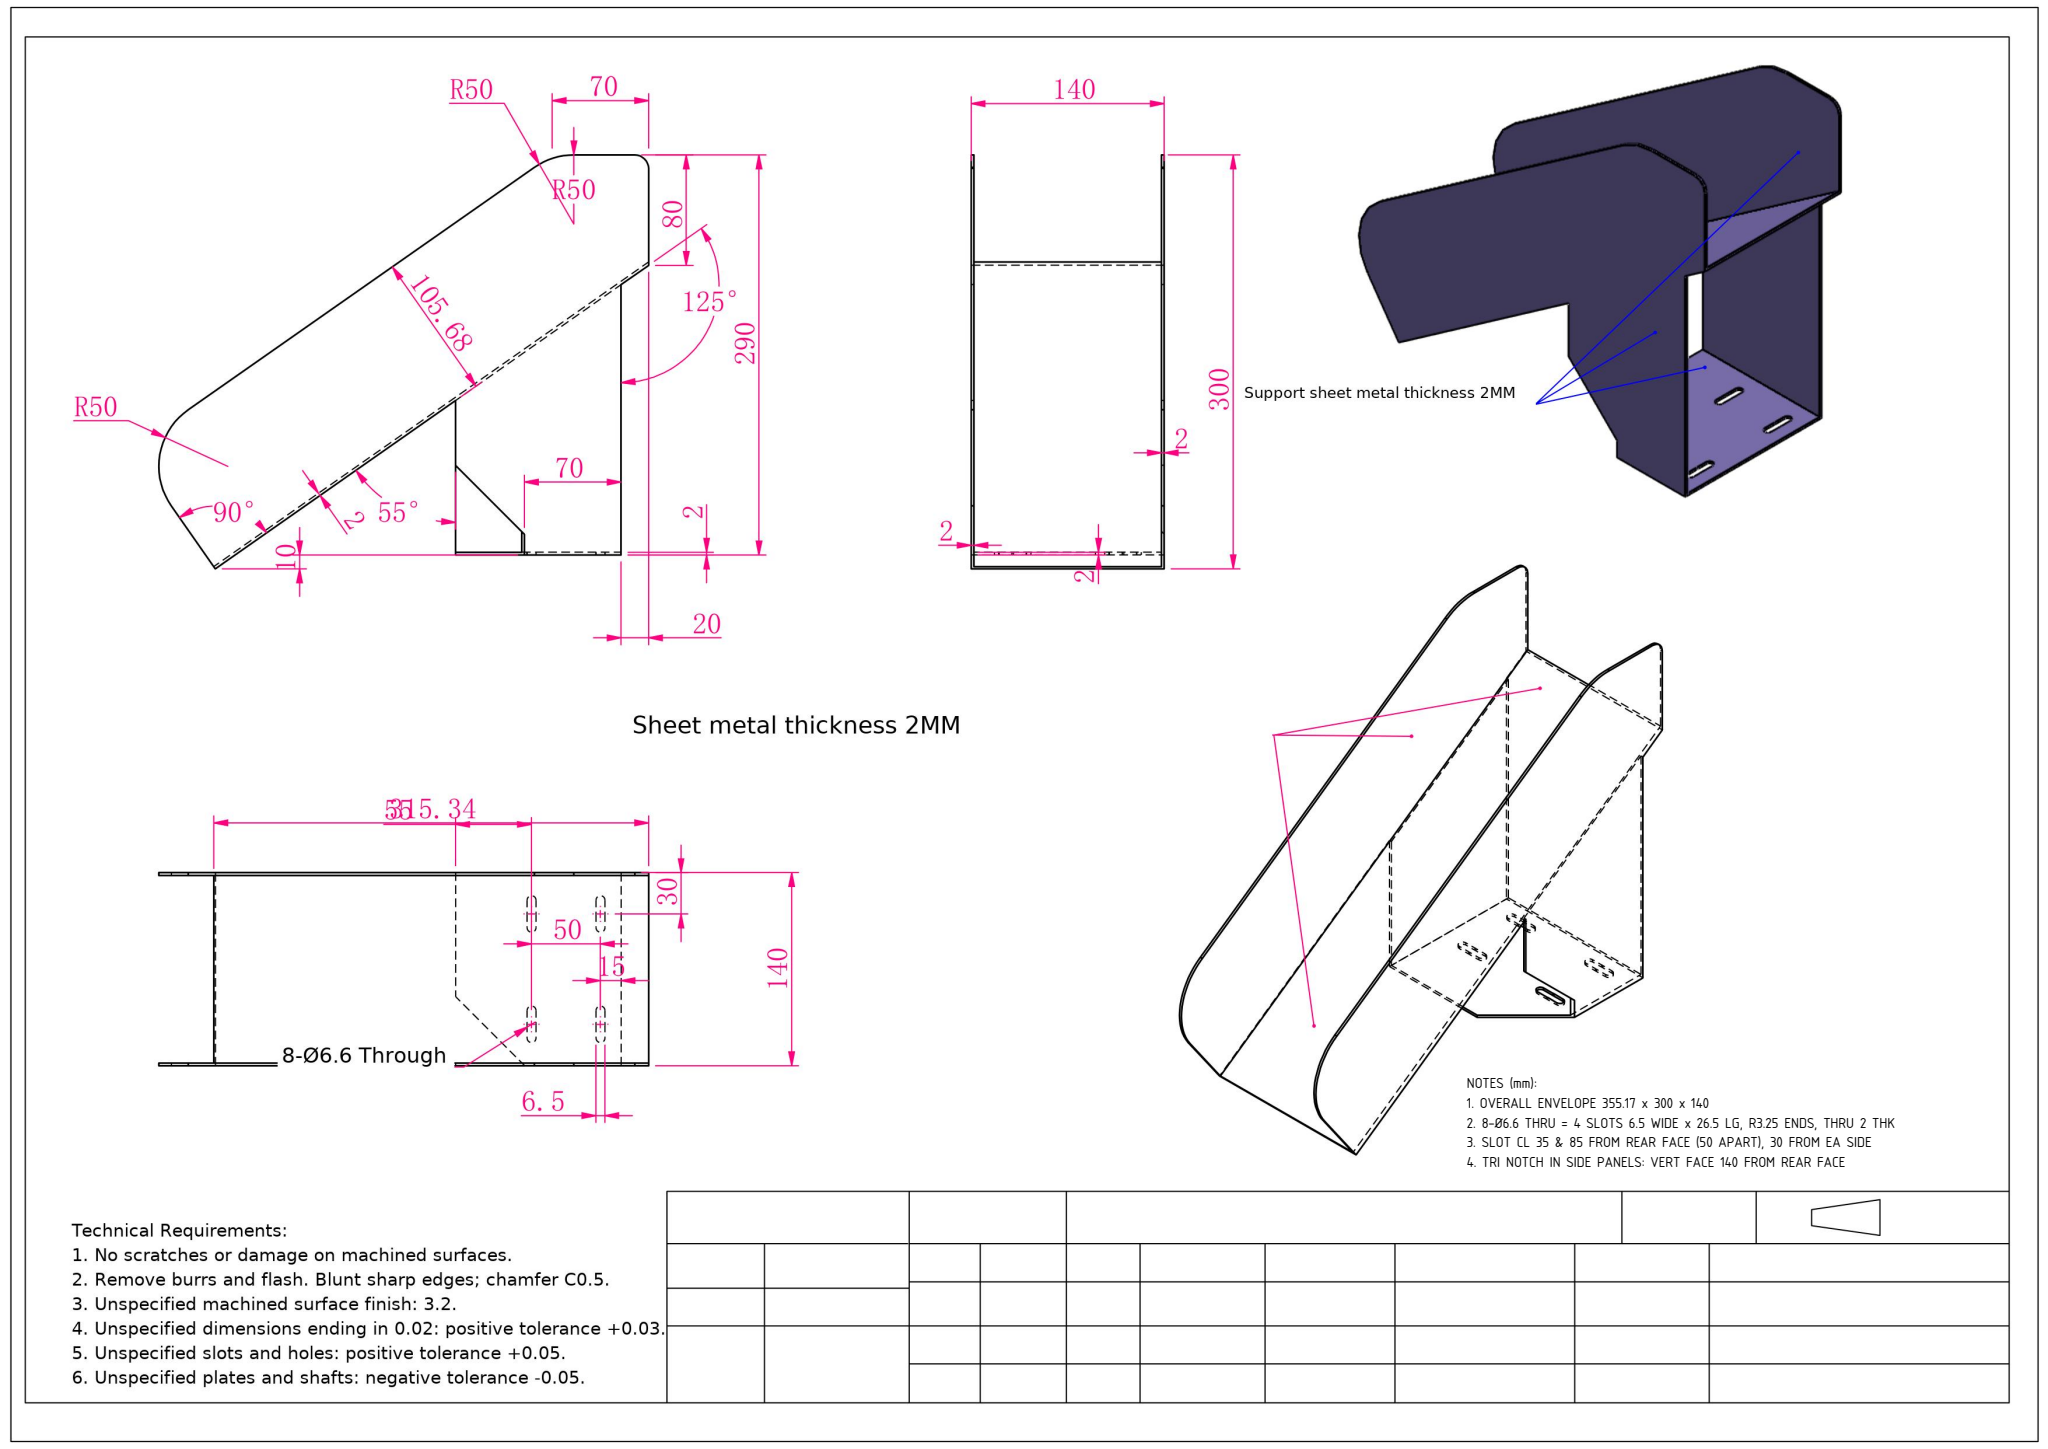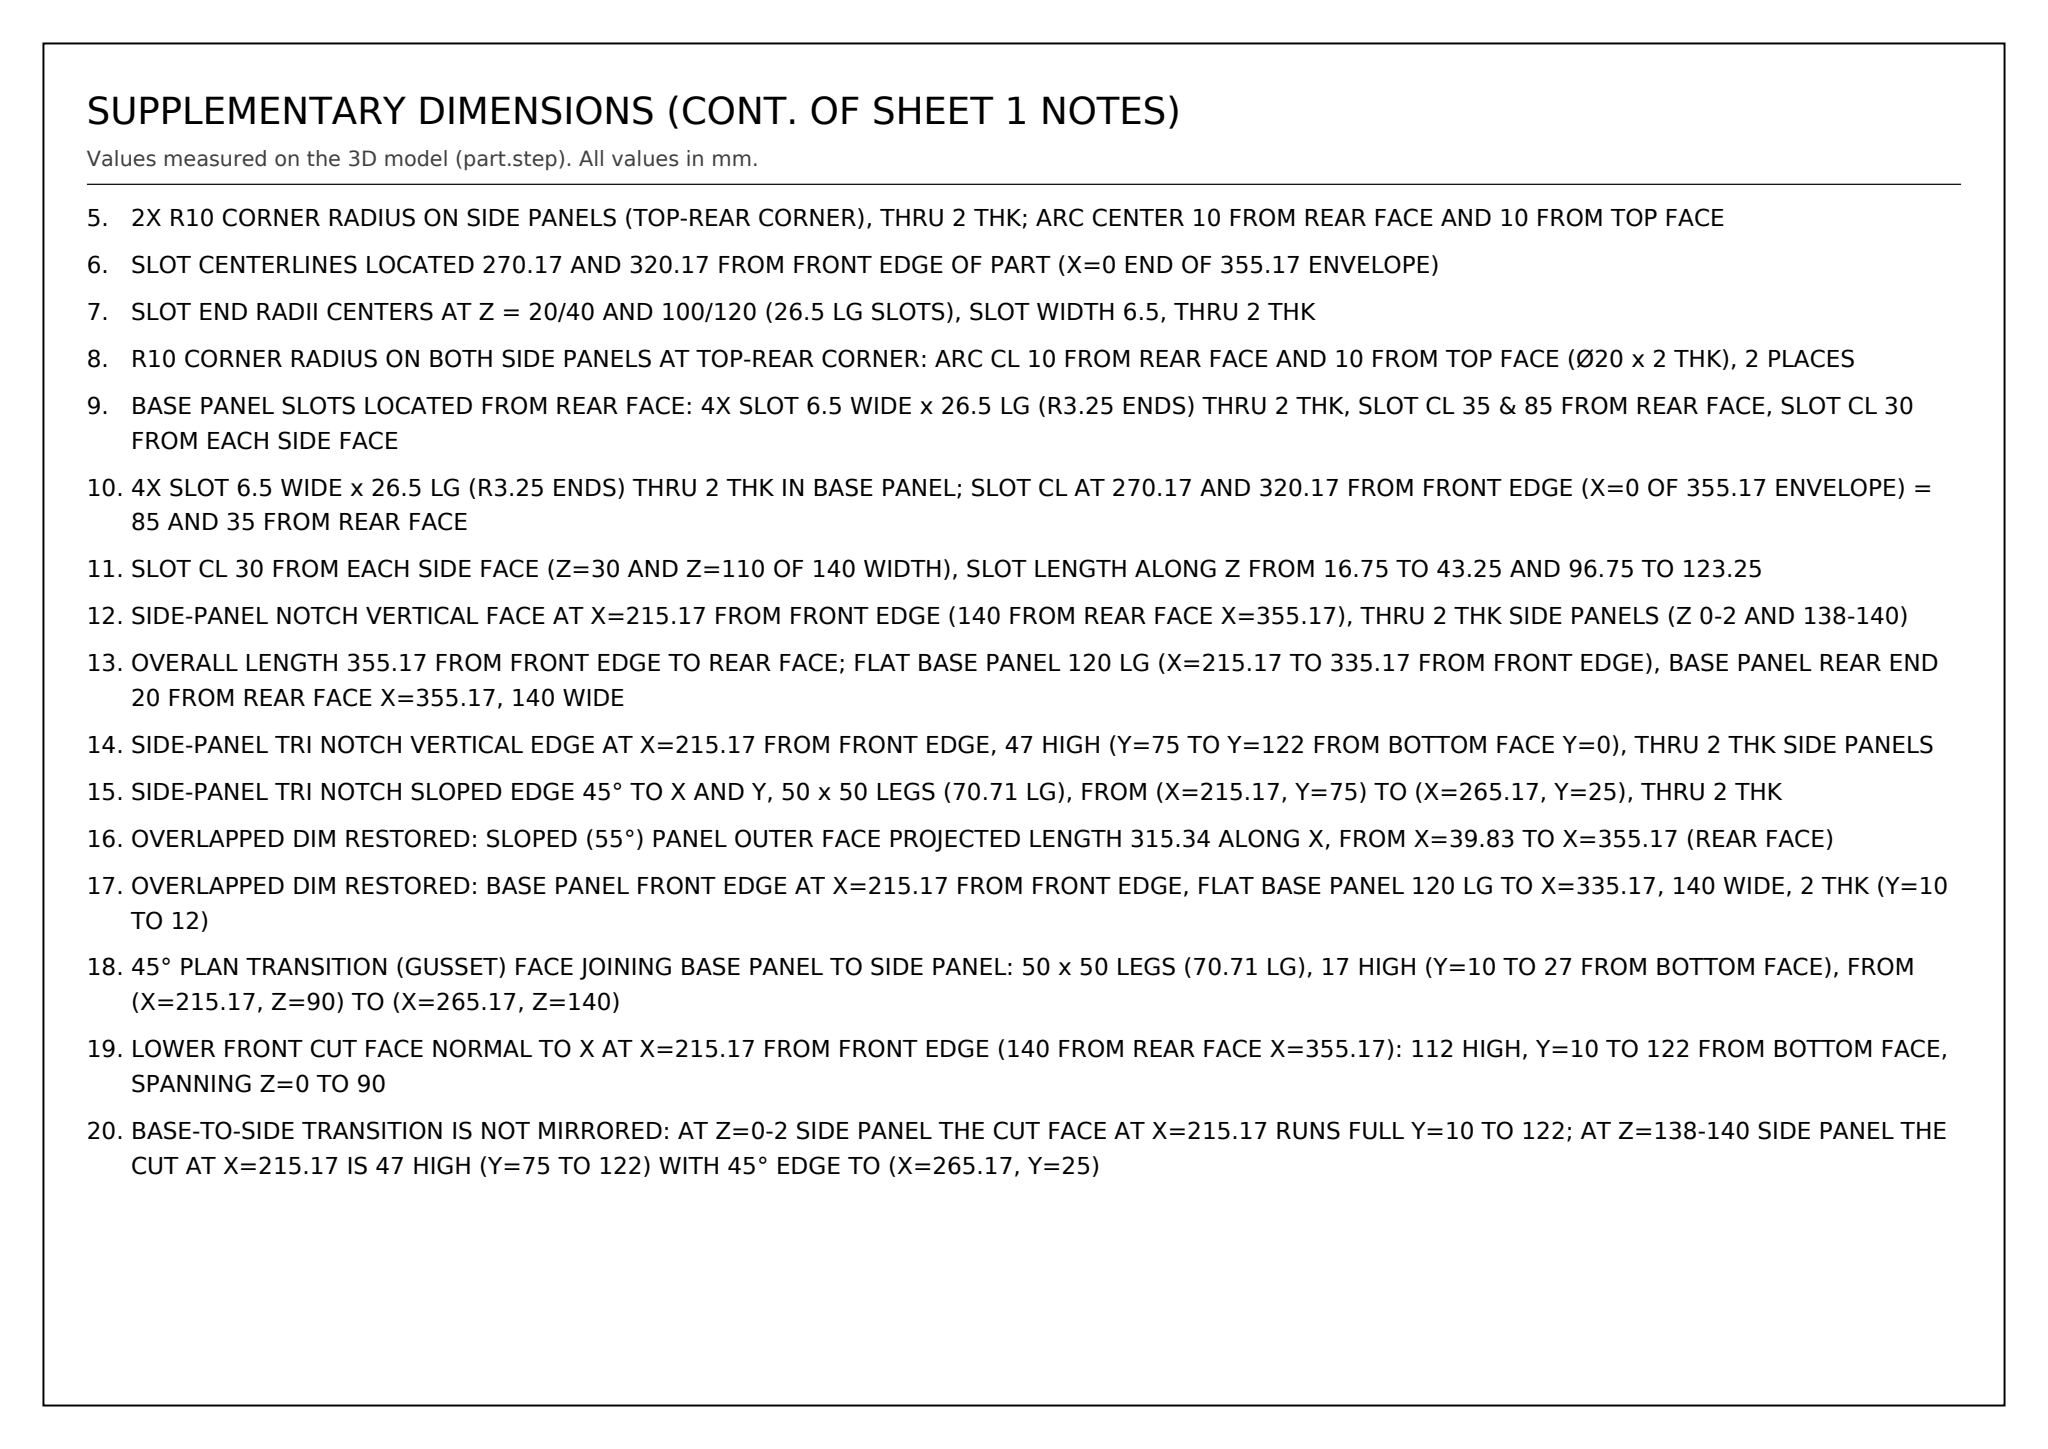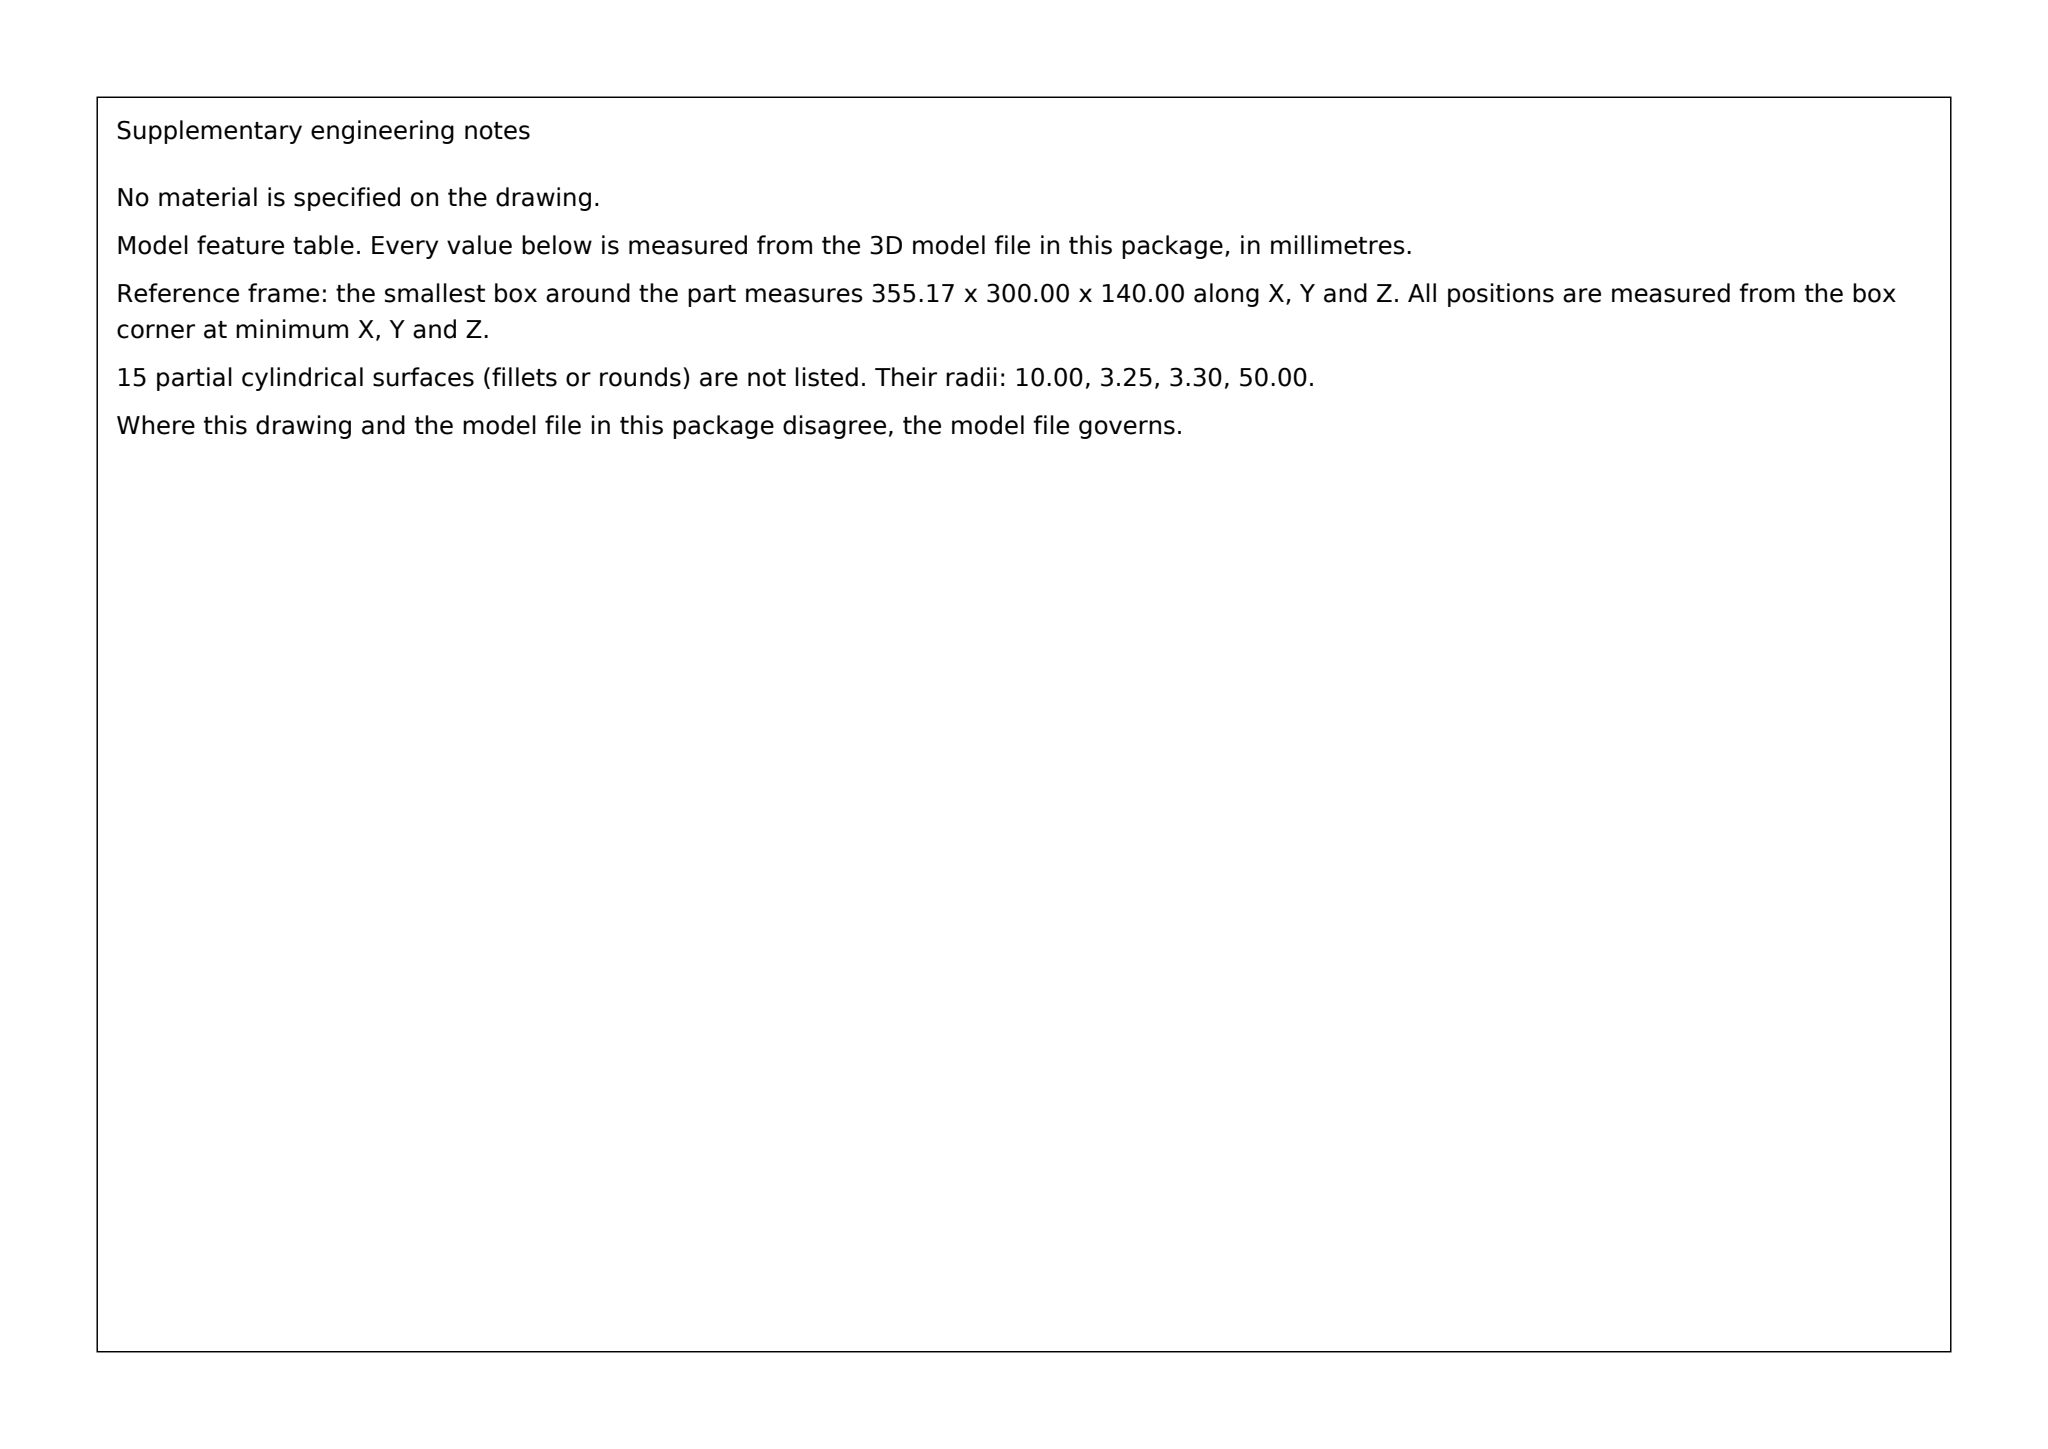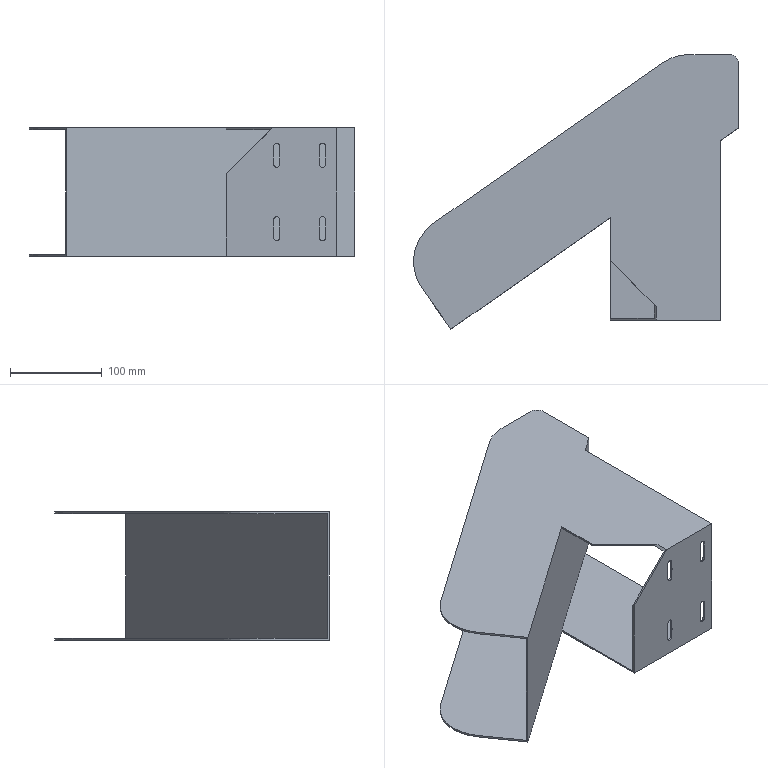Part | SolidWorks | mm | 1 solid | 65 faces | box 355.17 x 300 x 140 mm | volume 372082 mm3 | plane 37 | cylinder 28 | commonest cylinder face diameters 6.6 x12 6.5 x8 100 x6 20 x2
Drawing notes:
OVERALL ENVELOPE 355.17 x 300 x 140 | from the solid: bbox_xyz [355.173, 300.0, 140.0]
8-Ø6.6 THRU = 4 SLOTS 6.5 WIDE x 26.5 LG, R3.25 ENDS, THRU 2 THK | from the solid: Slot side planes x=266.92/273.42 & 316.92/323.42 (6.5 apart); Ø6.5 end arcs at z=20&40, 100&120 (20 betw ctrs) => 26.5 OAL; cyl length 2
SLOT CL 35 & 85 FROM REAR FACE (50 APART), 30 FROM EA SIDE | from the solid: Slot axes x=270.17 & 320.17 vs rear face x=355.17 => 85 & 35, 50 apart; z=30 & 110 vs sides z=0/140 => 30 ea side
TRI NOTCH IN SIDE PANELS: VERT FACE 140 FROM REAR FACE | from the solid: Plane normal x at 215.17 (2 off, one per 2 thk side panel z=0-2 & 138-140); 355.17-215.17=140
2X R10 CORNER RADIUS ON SIDE PANELS (TOP-REAR CORNER), THRU 2 THK; ARC CENTER 10 FROM REAR FACE AND 10 FROM TOP FACE | from the solid: cylinders: [20.0 dia, axis z, pos (345.17, 290.0), length 2.0, count 2] with bbox 355.173 x 300.0 x 140.0
SLOT CENTERLINES LOCATED 270.17 AND 320.17 FROM FRONT EDGE OF PART (X=0 END OF 355.17 ENVELOPE) | from the solid: cylinders 6.6 dia, axis y, at x = 270.17 and 320.17; bbox_xyz x = 355.173
SLOT END RADII CENTERS AT Z = 20/40 AND 100/120 (26.5 LG SLOTS), SLOT WIDTH 6.5, THRU 2 THK | from the solid: cylinders 6.5 dia, axis y, at z = 20.0, 40.0, 100.0, 120.0, length 2.0
R10 CORNER RADIUS ON BOTH SIDE PANELS AT TOP-REAR CORNER: ARC CL 10 FROM REAR FACE AND 10 FROM TOP FACE (Ø20 x 2 THK), 2 PLACES | from the solid: cylinders: [20.0,'z',[345.17,290.0],2.0, count 2] with bbox 355.173 x 300.0 x 140.0 (rear face x=355.17, top y=300)
BASE PANEL SLOTS LOCATED FROM REAR FACE: 4X SLOT 6.5 WIDE x 26.5 LG (R3.25 ENDS) THRU 2 THK, SLOT CL 35 & 85 FROM REAR FACE, SLOT CL 30 FROM EACH SIDE FACE | from the solid: cylinders Ø6.6 axis y at x=270.17 & 320.17, z=30 & 110; Ø6.5 end radii at z=20/40/100/120; planes x=266.92/273.42 and 316.92/323.42 (6.5 wide); bbox x=355.173, z=140
4X SLOT 6.5 WIDE x 26.5 LG (R3.25 ENDS) THRU 2 THK IN BASE PANEL; SLOT CL AT 270.17 AND 320.17 FROM FRONT EDGE (X=0 OF 355.17 ENVELOPE) = 85 AND 35 FROM REAR FACE | from the solid: cylinders dia 6.5 axis y at x=270.17 and x=320.17, z=20/40/100/120, length 2; axis_planes x=266.92/273.42/316.92/323.42 (6.5 slot width); bbox_xyz x=355.173
SLOT CL 30 FROM EACH SIDE FACE (Z=30 AND Z=110 OF 140 WIDTH), SLOT LENGTH ALONG Z FROM 16.75 TO 43.25 AND 96.75 TO 123.25 | from the solid: cylinders dia 6.5 at z=20/40 and z=100/120 with R3.25 ends; bbox_xyz z=140
SIDE-PANEL NOTCH VERTICAL FACE AT X=215.17 FROM FRONT EDGE (140 FROM REAR FACE X=355.17), THRU 2 THK SIDE PANELS (Z 0-2 AND 138-140) | from the solid: axis_planes x=215.17 (2); axis_planes z=0/2 and z=138/140; bbox_xyz x=355.173
OVERALL LENGTH 355.17 FROM FRONT EDGE TO REAR FACE; FLAT BASE PANEL 120 LG (X=215.17 TO 335.17 FROM FRONT EDGE), BASE PANEL REAR END 20 FROM REAR FACE X=355.17, 140 WIDE | from the solid: bbox_xyz [355.173,300,140]; axis plane y=10 extent x[215.2,335.2], z[0.0,140.0]; axis plane x=335.2 extent y[10,206]
SIDE-PANEL TRI NOTCH VERTICAL EDGE AT X=215.17 FROM FRONT EDGE, 47 HIGH (Y=75 TO Y=122 FROM BOTTOM FACE Y=0), THRU 2 THK SIDE PANELS | from the solid: axis plane x=215.2 extent y[75,122], z[138,140] (area 94); axis plane x=215.2 extent y[10,122], z[0,90]
SIDE-PANEL TRI NOTCH SLOPED EDGE 45° TO X AND Y, 50 x 50 LEGS (70.71 LG), FROM (X=215.17, Y=75) TO (X=265.17, Y=25), THRU 2 THK | from the solid: inclined plane angle_to_xyz_axes [45,45,90], bbox_from [215.2,25.0,138.0], size [50,50,2]
OVERLAPPED DIM RESTORED: SLOPED (55°) PANEL OUTER FACE PROJECTED LENGTH 315.34 ALONG X, FROM X=39.83 TO X=355.17 (REAR FACE) | from the solid: inclined_planes: angle_to_xyz [55,35,90], bbox_from [39.8,1.6,2.0], size [315.3,220.8,136.0]
OVERLAPPED DIM RESTORED: BASE PANEL FRONT EDGE AT X=215.17 FROM FRONT EDGE, FLAT BASE PANEL 120 LG TO X=335.17, 140 WIDE, 2 THK (Y=10 TO 12) | from the solid: axis_planes: y=10.0 extent x[215.2,335.2] z[0,140]; x=335.2 extent y[10,206] z[0,140]
45° PLAN TRANSITION (GUSSET) FACE JOINING BASE PANEL TO SIDE PANEL: 50 x 50 LEGS (70.71 LG), 17 HIGH (Y=10 TO 27 FROM BOTTOM FACE), FROM (X=215.17, Z=90) TO (X=265.17, Z=140) | from the solid: inclined_planes: angle_to_xyz [45,90,45], bbox_from [215.2,10.0,90.0], size [50,17,50]
LOWER FRONT CUT FACE NORMAL TO X AT X=215.17 FROM FRONT EDGE (140 FROM REAR FACE X=355.17): 112 HIGH, Y=10 TO 122 FROM BOTTOM FACE, SPANNING Z=0 TO 90 | from the solid: axis_planes: x=215.2 extent y[10.0,122.0] z[0.0,90.0]
BASE-TO-SIDE TRANSITION IS NOT MIRRORED: AT Z=0-2 SIDE PANEL THE CUT FACE AT X=215.17 RUNS FULL Y=10 TO 122; AT Z=138-140 SIDE PANEL THE CUT AT X=215.17 IS 47 HIGH (Y=75 TO 122) WITH 45° EDGE TO (X=265.17, Y=25) | from the solid: axis_planes: x=215.2 extent y[10,122] z[0,90] vs x=215.2 extent y[75,122] z[138,140]; inclined_planes angle [45,45,90] bbox_from [215.2,25.0,138.0] size [50,50,2]